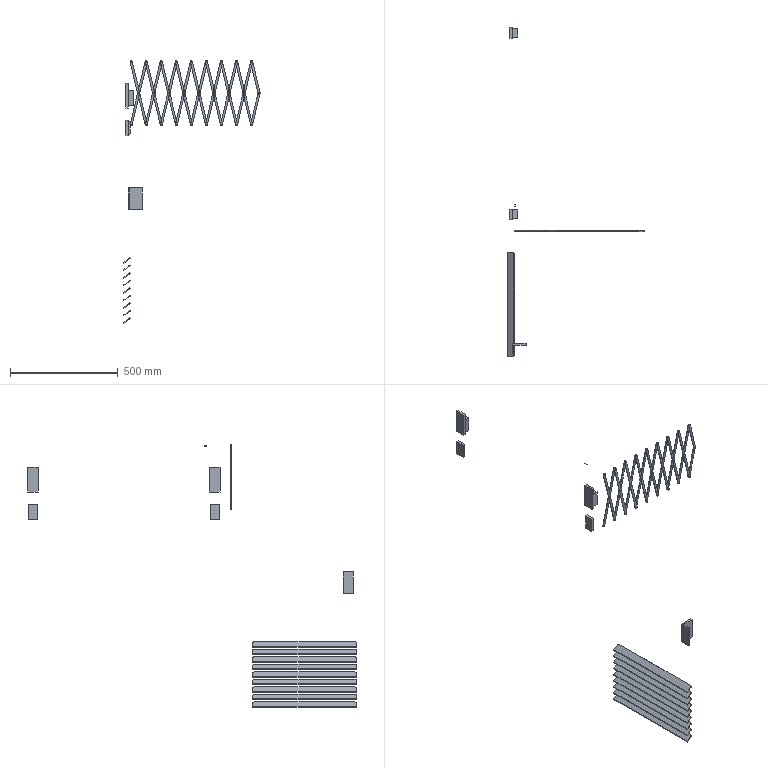Component | NX | Root-owned geometry | 35 solids | 287 faces | volume 1057930 mm3 | plane 180 | cylinder 107 | commonest cylinder face diameters 4 x53 10 x36 18 x18